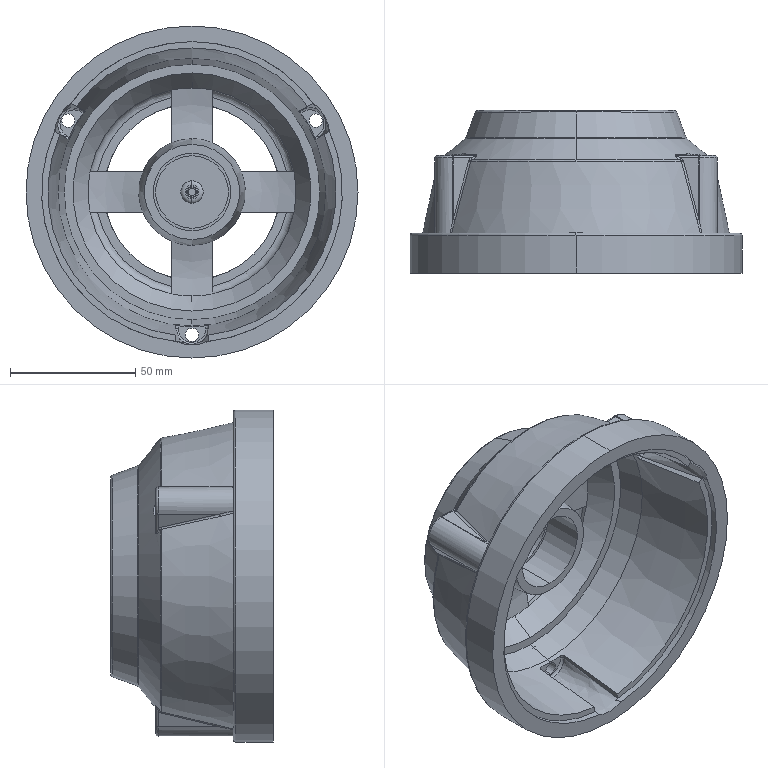Component | SolidWorks | Cache Festo AD85-2_Cache Festo AD85-1 | 1 solid | 200 faces | box 132.5 x 65 x 132.5 mm | volume 143976 mm3 | cylinder 62 | plane 52 | spline 40 | torus 31 | cone 15 | commonest cylinder face diameters 2 x12 11 x8 5.37 x6 14 x5 74 x4 42.5 x4 83 x4 120 x3